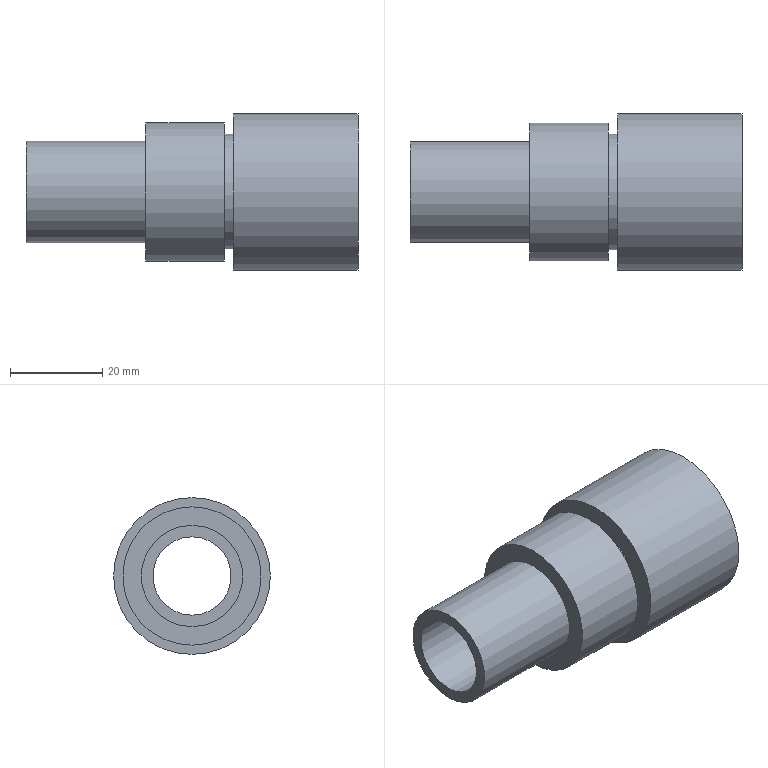Component | NX | SLEEVE | 1 solid | 14 faces | box 72 x 34 x 34 mm | volume 29705 mm3 | cylinder 7 | plane 7 | commonest cylinder face diameters 30 x1 22 x1 34 x1 17 x1 17.5 x1 25 x1 20 x1
STEP:
#1=CARTESIAN_POINT('',(0.,0.,0.));
#2=DIRECTION('',(0.,0.,1.));
#3=DIRECTION('',(1.,0.,0.));
#4=AXIS2_PLACEMENT_3D('',#1,#2,#3);
#5=CARTESIAN_POINT('',(21.,-0.,5.));
#6=VERTEX_POINT('',#5);
#7=CARTESIAN_POINT('',(21.,-0.,20.));
#8=DIRECTION('',(1.,0.,0.));
#9=DIRECTION('',(0.,0.,-1.));
#10=AXIS2_PLACEMENT_3D('',#7,#8,#9);
#11=CIRCLE('',#10,15.);
#12=CARTESIAN_POINT('',(40.,-0.,20.));
#13=DIRECTION('',(-1.,0.,0.));
#14=DIRECTION('',(0.,0.,1.));
#15=AXIS2_PLACEMENT_3D('',#12,#13,#14);
#16=CYLINDRICAL_SURFACE('',#15,15.);
#17=CARTESIAN_POINT('',(9.425,19.));
#18=DIRECTION('',(-1.,0.));
#19=VECTOR('',#18,1.);
#20=LINE('',#17,#19);
#21=(GEOMETRIC_REPRESENTATION_CONTEXT(2)PARAMETRIC_REPRESENTATION_CONTEXT()REPRESENTATION_CONTEXT('',''));
#22=DEFINITIONAL_REPRESENTATION('',(#20),#21);
#23=PCURVE('',#16,#22);
#24=CARTESIAN_POINT('',(21.,-0.,20.));
#25=DIRECTION('',(1.,0.,0.));
#26=DIRECTION('',(0.,0.,-1.));
#27=AXIS2_PLACEMENT_3D('',#24,#25,#26);
#28=PLANE('',#27);
#29=CARTESIAN_POINT('',(0.,0.));
#30=DIRECTION('',(1.,0.));
#31=AXIS2_PLACEMENT_2D('',#29,#30);
#32=CIRCLE('',#31,15.);
#33=(GEOMETRIC_REPRESENTATION_CONTEXT(2)PARAMETRIC_REPRESENTATION_CONTEXT()REPRESENTATION_CONTEXT('',''));
#34=DEFINITIONAL_REPRESENTATION('',(#32),#33);
#35=PCURVE('',#28,#34);
#36=SURFACE_CURVE('',#11,(#23,#35),.PCURVE_S1.);
#37=EDGE_CURVE('',#6,#6,#36,.T.);
#38=ORIENTED_EDGE('',*,*,#37,.T.);
#39=CARTESIAN_POINT('',(38.,-0.,5.));
#40=VERTEX_POINT('',#39);
#41=CARTESIAN_POINT('',(38.,-0.,5.));
#42=CARTESIAN_POINT('',(21.,-0.,5.));
#43=B_SPLINE_CURVE_WITH_KNOTS('',1,(#41,#42),.UNSPECIFIED.,.F.,.F.,(2,2),(2.,19.),.PIECEWISE_BEZIER_KNOTS.);
#44=CARTESIAN_POINT('',(3.142,0.));
#45=DIRECTION('',(0.,1.));
#46=VECTOR('',#45,1.);
#47=LINE('',#44,#46);
#48=(GEOMETRIC_REPRESENTATION_CONTEXT(2)PARAMETRIC_REPRESENTATION_CONTEXT()REPRESENTATION_CONTEXT('',''));
#49=DEFINITIONAL_REPRESENTATION('',(#47),#48);
#50=PCURVE('',#16,#49);
#51=CARTESIAN_POINT('',(9.425,0.));
#52=DIRECTION('',(0.,1.));
#53=VECTOR('',#52,1.);
#54=LINE('',#51,#53);
#55=(GEOMETRIC_REPRESENTATION_CONTEXT(2)PARAMETRIC_REPRESENTATION_CONTEXT()REPRESENTATION_CONTEXT('',''));
#56=DEFINITIONAL_REPRESENTATION('',(#54),#55);
#57=PCURVE('',#16,#56);
#58=SEAM_CURVE('',#43,(#50,#57),.PCURVE_S1.);
#59=EDGE_CURVE('',#40,#6,#58,.T.);
#60=ORIENTED_EDGE('',*,*,#59,.F.);
#61=CARTESIAN_POINT('',(38.,-0.,20.));
#62=DIRECTION('',(1.,0.,0.));
#63=DIRECTION('',(0.,0.,-1.));
#64=AXIS2_PLACEMENT_3D('',#61,#62,#63);
#65=CIRCLE('',#64,15.);
#66=CARTESIAN_POINT('',(9.425,2.));
#67=DIRECTION('',(-1.,0.));
#68=VECTOR('',#67,1.);
#69=LINE('',#66,#68);
#70=(GEOMETRIC_REPRESENTATION_CONTEXT(2)PARAMETRIC_REPRESENTATION_CONTEXT()REPRESENTATION_CONTEXT('',''));
#71=DEFINITIONAL_REPRESENTATION('',(#69),#70);
#72=PCURVE('',#16,#71);
#73=CARTESIAN_POINT('',(38.,-0.,20.));
#74=DIRECTION('',(-1.,0.,0.));
#75=DIRECTION('',(0.,0.,1.));
#76=AXIS2_PLACEMENT_3D('',#73,#74,#75);
#77=PLANE('',#76);
#78=CARTESIAN_POINT('',(-15.,0.));
#79=CARTESIAN_POINT('',(-15.,25.981));
#80=CARTESIAN_POINT('',(7.5,12.99));
#81=CARTESIAN_POINT('',(30.,0.));
#82=CARTESIAN_POINT('',(7.5,-12.99));
#83=CARTESIAN_POINT('',(-15.,-25.981));
#84=CARTESIAN_POINT('',(-15.,0.));
#85=(BOUNDED_CURVE()B_SPLINE_CURVE(2,(#78,#79,#80,#81,#82,#83,#84),.UNSPECIFIED.,.T.,.F.)B_SPLINE_CURVE_WITH_KNOTS((1,2,2,2,2,1),(-2.094,0.,2.094,4.189,6.283,8.378),.UNSPECIFIED.)CURVE()GEOMETRIC_REPRESENTATION_ITEM()RATIONAL_B_SPLINE_CURVE((1.,0.5,1.,0.5,1.,0.5,1.))REPRESENTATION_ITEM(''));
#86=(GEOMETRIC_REPRESENTATION_CONTEXT(2)PARAMETRIC_REPRESENTATION_CONTEXT()REPRESENTATION_CONTEXT('',''));
#87=DEFINITIONAL_REPRESENTATION('',(#85),#86);
#88=PCURVE('',#77,#87);
#89=SURFACE_CURVE('',#65,(#72,#88),.PCURVE_S1.);
#90=EDGE_CURVE('',#40,#40,#89,.T.);
#91=ORIENTED_EDGE('',*,*,#90,.F.);
#92=ORIENTED_EDGE('',*,*,#59,.T.);
#93=EDGE_LOOP('',(#38,#60,#91,#92));
#94=FACE_BOUND('',#93,.T.);
#95=ADVANCED_FACE('',(#94),#16,.T.);
#96=CARTESIAN_POINT('',(21.,-0.,9.));
#97=VERTEX_POINT('',#96);
#98=CARTESIAN_POINT('',(21.,-0.,20.));
#99=DIRECTION('',(1.,0.,0.));
#100=DIRECTION('',(0.,0.,-1.));
#101=AXIS2_PLACEMENT_3D('',#98,#99,#100);
#102=CIRCLE('',#101,11.);
#103=CARTESIAN_POINT('',(21.,-0.,20.));
#104=DIRECTION('',(-1.,0.,0.));
#105=DIRECTION('',(0.,0.,1.));
#106=AXIS2_PLACEMENT_3D('',#103,#104,#105);
#107=CYLINDRICAL_SURFACE('',#106,11.);
#108=CARTESIAN_POINT('',(9.425,0.));
#109=DIRECTION('',(-1.,0.));
#110=VECTOR('',#109,1.);
#111=LINE('',#108,#110);
#112=(GEOMETRIC_REPRESENTATION_CONTEXT(2)PARAMETRIC_REPRESENTATION_CONTEXT()REPRESENTATION_CONTEXT('',''));
#113=DEFINITIONAL_REPRESENTATION('',(#111),#112);
#114=PCURVE('',#107,#113);
#115=CARTESIAN_POINT('',(0.,0.));
#116=DIRECTION('',(1.,0.));
#117=AXIS2_PLACEMENT_2D('',#115,#116);
#118=CIRCLE('',#117,11.);
#119=(GEOMETRIC_REPRESENTATION_CONTEXT(2)PARAMETRIC_REPRESENTATION_CONTEXT()REPRESENTATION_CONTEXT('',''));
#120=DEFINITIONAL_REPRESENTATION('',(#118),#119);
#121=PCURVE('',#28,#120);
#122=SURFACE_CURVE('',#102,(#114,#121),.PCURVE_S1.);
#123=EDGE_CURVE('',#97,#97,#122,.T.);
#124=ORIENTED_EDGE('',*,*,#123,.F.);
#125=CARTESIAN_POINT('',(-5.,-0.,9.));
#126=VERTEX_POINT('',#125);
#127=CARTESIAN_POINT('',(21.,-0.,9.));
#128=CARTESIAN_POINT('',(-5.,-0.,9.));
#129=B_SPLINE_CURVE_WITH_KNOTS('',1,(#127,#128),.UNSPECIFIED.,.F.,.F.,(2,2),(0.,26.),.PIECEWISE_BEZIER_KNOTS.);
#130=CARTESIAN_POINT('',(9.425,0.));
#131=DIRECTION('',(0.,1.));
#132=VECTOR('',#131,1.);
#133=LINE('',#130,#132);
#134=(GEOMETRIC_REPRESENTATION_CONTEXT(2)PARAMETRIC_REPRESENTATION_CONTEXT()REPRESENTATION_CONTEXT('',''));
#135=DEFINITIONAL_REPRESENTATION('',(#133),#134);
#136=PCURVE('',#107,#135);
#137=CARTESIAN_POINT('',(3.142,0.));
#138=DIRECTION('',(0.,1.));
#139=VECTOR('',#138,1.);
#140=LINE('',#137,#139);
#141=(GEOMETRIC_REPRESENTATION_CONTEXT(2)PARAMETRIC_REPRESENTATION_CONTEXT()REPRESENTATION_CONTEXT('',''));
#142=DEFINITIONAL_REPRESENTATION('',(#140),#141);
#143=PCURVE('',#107,#142);
#144=SEAM_CURVE('',#129,(#136,#143),.PCURVE_S1.);
#145=EDGE_CURVE('',#97,#126,#144,.T.);
#146=ORIENTED_EDGE('',*,*,#145,.T.);
#147=CARTESIAN_POINT('',(-5.,-0.,20.));
#148=DIRECTION('',(1.,0.,0.));
#149=DIRECTION('',(0.,0.,-1.));
#150=AXIS2_PLACEMENT_3D('',#147,#148,#149);
#151=CIRCLE('',#150,11.);
#152=CARTESIAN_POINT('',(9.425,26.));
#153=DIRECTION('',(-1.,0.));
#154=VECTOR('',#153,1.);
#155=LINE('',#152,#154);
#156=(GEOMETRIC_REPRESENTATION_CONTEXT(2)PARAMETRIC_REPRESENTATION_CONTEXT()REPRESENTATION_CONTEXT('',''));
#157=DEFINITIONAL_REPRESENTATION('',(#155),#156);
#158=PCURVE('',#107,#157);
#159=CARTESIAN_POINT('',(-5.,-0.,20.));
#160=DIRECTION('',(1.,0.,0.));
#161=DIRECTION('',(0.,0.,-1.));
#162=AXIS2_PLACEMENT_3D('',#159,#160,#161);
#163=PLANE('',#162);
#164=CARTESIAN_POINT('',(0.,0.));
#165=DIRECTION('',(1.,0.));
#166=AXIS2_PLACEMENT_2D('',#164,#165);
#167=CIRCLE('',#166,11.);
#168=(GEOMETRIC_REPRESENTATION_CONTEXT(2)PARAMETRIC_REPRESENTATION_CONTEXT()REPRESENTATION_CONTEXT('',''));
#169=DEFINITIONAL_REPRESENTATION('',(#167),#168);
#170=PCURVE('',#163,#169);
#171=SURFACE_CURVE('',#151,(#158,#170),.PCURVE_S1.);
#172=EDGE_CURVE('',#126,#126,#171,.T.);
#173=ORIENTED_EDGE('',*,*,#172,.T.);
#174=ORIENTED_EDGE('',*,*,#145,.F.);
#175=EDGE_LOOP('',(#124,#146,#173,#174));
#176=FACE_BOUND('',#175,.T.);
#177=ADVANCED_FACE('',(#176),#107,.T.);
#178=CARTESIAN_POINT('',(-5.,-0.,11.5));
#179=VERTEX_POINT('',#178);
#180=CARTESIAN_POINT('',(-5.,-0.,20.));
#181=DIRECTION('',(1.,0.,0.));
#182=DIRECTION('',(0.,0.,-1.));
#183=AXIS2_PLACEMENT_3D('',#180,#181,#182);
#184=CIRCLE('',#183,8.5);
#185=CARTESIAN_POINT('',(0.,0.));
#186=DIRECTION('',(1.,0.));
#187=AXIS2_PLACEMENT_2D('',#185,#186);
#188=CIRCLE('',#187,8.5);
#189=(GEOMETRIC_REPRESENTATION_CONTEXT(2)PARAMETRIC_REPRESENTATION_CONTEXT()REPRESENTATION_CONTEXT('',''));
#190=DEFINITIONAL_REPRESENTATION('',(#188),#189);
#191=PCURVE('',#163,#190);
#192=CARTESIAN_POINT('',(-5.,-0.,20.));
#193=DIRECTION('',(1.,0.,0.));
#194=DIRECTION('',(0.,0.,-1.));
#195=AXIS2_PLACEMENT_3D('',#192,#193,#194);
#196=CYLINDRICAL_SURFACE('',#195,8.5);
#197=CARTESIAN_POINT('',(0.,0.));
#198=DIRECTION('',(1.,0.));
#199=VECTOR('',#198,1.);
#200=LINE('',#197,#199);
#201=(GEOMETRIC_REPRESENTATION_CONTEXT(2)PARAMETRIC_REPRESENTATION_CONTEXT()REPRESENTATION_CONTEXT('',''));
#202=DEFINITIONAL_REPRESENTATION('',(#200),#201);
#203=PCURVE('',#196,#202);
#204=SURFACE_CURVE('',#184,(#191,#203),.PCURVE_S1.);
#205=EDGE_CURVE('',#179,#179,#204,.T.);
#206=ORIENTED_EDGE('',*,*,#205,.T.);
#207=EDGE_LOOP('',(#206));
#208=FACE_BOUND('',#207,.T.);
#209=ORIENTED_EDGE('',*,*,#172,.F.);
#210=EDGE_LOOP('',(#209));
#211=FACE_BOUND('',#210,.T.);
#212=ADVANCED_FACE('',(#208,#211),#163,.F.);
#213=ORIENTED_EDGE('',*,*,#123,.T.);
#214=EDGE_LOOP('',(#213));
#215=FACE_BOUND('',#214,.T.);
#216=ORIENTED_EDGE('',*,*,#37,.F.);
#217=EDGE_LOOP('',(#216));
#218=FACE_BOUND('',#217,.T.);
#219=ADVANCED_FACE('',(#215,#218),#28,.F.);
#220=CARTESIAN_POINT('',(67.,-0.,3.));
#221=VERTEX_POINT('',#220);
#222=CARTESIAN_POINT('',(67.,-0.,20.));
#223=DIRECTION('',(1.,0.,0.));
#224=DIRECTION('',(0.,0.,-1.));
#225=AXIS2_PLACEMENT_3D('',#222,#223,#224);
#226=CIRCLE('',#225,17.);
#227=CARTESIAN_POINT('',(67.,-0.,20.));
#228=DIRECTION('',(-1.,0.,0.));
#229=DIRECTION('',(0.,0.,1.));
#230=AXIS2_PLACEMENT_3D('',#227,#228,#229);
#231=CYLINDRICAL_SURFACE('',#230,17.);
#232=CARTESIAN_POINT('',(9.425,0.));
#233=DIRECTION('',(-1.,0.));
#234=VECTOR('',#233,1.);
#235=LINE('',#232,#234);
#236=(GEOMETRIC_REPRESENTATION_CONTEXT(2)PARAMETRIC_REPRESENTATION_CONTEXT()REPRESENTATION_CONTEXT('',''));
#237=DEFINITIONAL_REPRESENTATION('',(#235),#236);
#238=PCURVE('',#231,#237);
#239=CARTESIAN_POINT('',(67.,-0.,20.));
#240=DIRECTION('',(1.,0.,0.));
#241=DIRECTION('',(0.,0.,-1.));
#242=AXIS2_PLACEMENT_3D('',#239,#240,#241);
#243=PLANE('',#242);
#244=CARTESIAN_POINT('',(0.,0.));
#245=DIRECTION('',(1.,0.));
#246=AXIS2_PLACEMENT_2D('',#244,#245);
#247=CIRCLE('',#246,17.);
#248=(GEOMETRIC_REPRESENTATION_CONTEXT(2)PARAMETRIC_REPRESENTATION_CONTEXT()REPRESENTATION_CONTEXT('',''));
#249=DEFINITIONAL_REPRESENTATION('',(#247),#248);
#250=PCURVE('',#243,#249);
#251=SURFACE_CURVE('',#226,(#238,#250),.PCURVE_S1.);
#252=EDGE_CURVE('',#221,#221,#251,.T.);
#253=ORIENTED_EDGE('',*,*,#252,.F.);
#254=CARTESIAN_POINT('',(40.,-0.,3.));
#255=VERTEX_POINT('',#254);
#256=CARTESIAN_POINT('',(67.,-0.,3.));
#257=CARTESIAN_POINT('',(40.,-0.,3.));
#258=B_SPLINE_CURVE_WITH_KNOTS('',1,(#256,#257),.UNSPECIFIED.,.F.,.F.,(2,2),(0.,27.),.PIECEWISE_BEZIER_KNOTS.);
#259=CARTESIAN_POINT('',(9.425,0.));
#260=DIRECTION('',(0.,1.));
#261=VECTOR('',#260,1.);
#262=LINE('',#259,#261);
#263=(GEOMETRIC_REPRESENTATION_CONTEXT(2)PARAMETRIC_REPRESENTATION_CONTEXT()REPRESENTATION_CONTEXT('',''));
#264=DEFINITIONAL_REPRESENTATION('',(#262),#263);
#265=PCURVE('',#231,#264);
#266=CARTESIAN_POINT('',(3.142,0.));
#267=DIRECTION('',(0.,1.));
#268=VECTOR('',#267,1.);
#269=LINE('',#266,#268);
#270=(GEOMETRIC_REPRESENTATION_CONTEXT(2)PARAMETRIC_REPRESENTATION_CONTEXT()REPRESENTATION_CONTEXT('',''));
#271=DEFINITIONAL_REPRESENTATION('',(#269),#270);
#272=PCURVE('',#231,#271);
#273=SEAM_CURVE('',#258,(#265,#272),.PCURVE_S1.);
#274=EDGE_CURVE('',#221,#255,#273,.T.);
#275=ORIENTED_EDGE('',*,*,#274,.T.);
#276=CARTESIAN_POINT('',(40.,-0.,20.));
#277=DIRECTION('',(1.,0.,0.));
#278=DIRECTION('',(0.,0.,-1.));
#279=AXIS2_PLACEMENT_3D('',#276,#277,#278);
#280=CIRCLE('',#279,17.);
#281=CARTESIAN_POINT('',(9.425,27.));
#282=DIRECTION('',(-1.,0.));
#283=VECTOR('',#282,1.);
#284=LINE('',#281,#283);
#285=(GEOMETRIC_REPRESENTATION_CONTEXT(2)PARAMETRIC_REPRESENTATION_CONTEXT()REPRESENTATION_CONTEXT('',''));
#286=DEFINITIONAL_REPRESENTATION('',(#284),#285);
#287=PCURVE('',#231,#286);
#288=CARTESIAN_POINT('',(40.,-0.,20.));
#289=DIRECTION('',(1.,0.,0.));
#290=DIRECTION('',(0.,0.,-1.));
#291=AXIS2_PLACEMENT_3D('',#288,#289,#290);
#292=PLANE('',#291);
#293=CARTESIAN_POINT('',(0.,0.));
#294=DIRECTION('',(1.,0.));
#295=AXIS2_PLACEMENT_2D('',#293,#294);
#296=CIRCLE('',#295,17.);
#297=(GEOMETRIC_REPRESENTATION_CONTEXT(2)PARAMETRIC_REPRESENTATION_CONTEXT()REPRESENTATION_CONTEXT('',''));
#298=DEFINITIONAL_REPRESENTATION('',(#296),#297);
#299=PCURVE('',#292,#298);
#300=SURFACE_CURVE('',#280,(#287,#299),.PCURVE_S1.);
#301=EDGE_CURVE('',#255,#255,#300,.T.);
#302=ORIENTED_EDGE('',*,*,#301,.T.);
#303=ORIENTED_EDGE('',*,*,#274,.F.);
#304=EDGE_LOOP('',(#253,#275,#302,#303));
#305=FACE_BOUND('',#304,.T.);
#306=ADVANCED_FACE('',(#305),#231,.T.);
#307=CARTESIAN_POINT('',(67.,-0.,10.));
#308=VERTEX_POINT('',#307);
#309=CARTESIAN_POINT('',(67.,-0.,20.));
#310=DIRECTION('',(1.,0.,0.));
#311=DIRECTION('',(0.,0.,-1.));
#312=AXIS2_PLACEMENT_3D('',#309,#310,#311);
#313=CIRCLE('',#312,10.);
#314=CARTESIAN_POINT('',(0.,0.));
#315=DIRECTION('',(1.,0.));
#316=AXIS2_PLACEMENT_2D('',#314,#315);
#317=CIRCLE('',#316,10.);
#318=(GEOMETRIC_REPRESENTATION_CONTEXT(2)PARAMETRIC_REPRESENTATION_CONTEXT()REPRESENTATION_CONTEXT('',''));
#319=DEFINITIONAL_REPRESENTATION('',(#317),#318);
#320=PCURVE('',#243,#319);
#321=CARTESIAN_POINT('',(52.,-0.,20.));
#322=DIRECTION('',(1.,0.,0.));
#323=DIRECTION('',(0.,0.,-1.));
#324=AXIS2_PLACEMENT_3D('',#321,#322,#323);
#325=CYLINDRICAL_SURFACE('',#324,10.);
#326=CARTESIAN_POINT('',(0.,15.));
#327=DIRECTION('',(1.,0.));
#328=VECTOR('',#327,1.);
#329=LINE('',#326,#328);
#330=(GEOMETRIC_REPRESENTATION_CONTEXT(2)PARAMETRIC_REPRESENTATION_CONTEXT()REPRESENTATION_CONTEXT('',''));
#331=DEFINITIONAL_REPRESENTATION('',(#329),#330);
#332=PCURVE('',#325,#331);
#333=SURFACE_CURVE('',#313,(#320,#332),.PCURVE_S1.);
#334=EDGE_CURVE('',#308,#308,#333,.T.);
#335=ORIENTED_EDGE('',*,*,#334,.F.);
#336=EDGE_LOOP('',(#335));
#337=FACE_BOUND('',#336,.T.);
#338=ORIENTED_EDGE('',*,*,#252,.T.);
#339=EDGE_LOOP('',(#338));
#340=FACE_BOUND('',#339,.T.);
#341=ADVANCED_FACE('',(#337,#340),#243,.T.);
#342=ORIENTED_EDGE('',*,*,#301,.F.);
#343=EDGE_LOOP('',(#342));
#344=FACE_BOUND('',#343,.T.);
#345=CARTESIAN_POINT('',(40.,-0.,32.5));
#346=VERTEX_POINT('',#345);
#347=CARTESIAN_POINT('',(40.,-0.,20.));
#348=DIRECTION('',(1.,0.,0.));
#349=DIRECTION('',(0.,0.,1.));
#350=AXIS2_PLACEMENT_3D('',#347,#348,#349);
#351=CIRCLE('',#350,12.5);
#352=CARTESIAN_POINT('',(0.,0.));
#353=DIRECTION('',(-1.,0.));
#354=AXIS2_PLACEMENT_2D('',#352,#353);
#355=CIRCLE('',#354,12.5);
#356=(GEOMETRIC_REPRESENTATION_CONTEXT(2)PARAMETRIC_REPRESENTATION_CONTEXT()REPRESENTATION_CONTEXT('',''));
#357=DEFINITIONAL_REPRESENTATION('',(#355),#356);
#358=PCURVE('',#292,#357);
#359=CARTESIAN_POINT('',(40.,-0.,20.));
#360=DIRECTION('',(-1.,0.,0.));
#361=DIRECTION('',(0.,0.,1.));
#362=AXIS2_PLACEMENT_3D('',#359,#360,#361);
#363=CYLINDRICAL_SURFACE('',#362,12.5);
#364=CARTESIAN_POINT('',(6.283,0.));
#365=DIRECTION('',(-1.,0.));
#366=VECTOR('',#365,1.);
#367=LINE('',#364,#366);
#368=(GEOMETRIC_REPRESENTATION_CONTEXT(2)PARAMETRIC_REPRESENTATION_CONTEXT()REPRESENTATION_CONTEXT('',''));
#369=DEFINITIONAL_REPRESENTATION('',(#367),#368);
#370=PCURVE('',#363,#369);
#371=SURFACE_CURVE('',#351,(#358,#370),.PCURVE_S1.);
#372=EDGE_CURVE('',#346,#346,#371,.T.);
#373=ORIENTED_EDGE('',*,*,#372,.T.);
#374=EDGE_LOOP('',(#373));
#375=FACE_BOUND('',#374,.T.);
#376=ADVANCED_FACE('',(#344,#375),#292,.F.);
#377=CARTESIAN_POINT('',(49.,-0.,11.5));
#378=VERTEX_POINT('',#377);
#379=CARTESIAN_POINT('',(49.,-0.,28.5));
#380=VERTEX_POINT('',#379);
#381=CARTESIAN_POINT('',(49.,-0.,20.));
#382=DIRECTION('',(1.,0.,0.));
#383=DIRECTION('',(0.,0.,1.));
#384=AXIS2_PLACEMENT_3D('',#381,#382,#383);
#385=CIRCLE('',#384,8.5);
#386=CARTESIAN_POINT('',(-3.142,54.));
#387=DIRECTION('',(1.,0.));
#388=VECTOR('',#387,1.);
#389=LINE('',#386,#388);
#390=(GEOMETRIC_REPRESENTATION_CONTEXT(2)PARAMETRIC_REPRESENTATION_CONTEXT()REPRESENTATION_CONTEXT('',''));
#391=DEFINITIONAL_REPRESENTATION('',(#389),#390);
#392=PCURVE('',#196,#391);
#393=CARTESIAN_POINT('',(49.,-0.,20.));
#394=DIRECTION('',(-1.,0.,0.));
#395=DIRECTION('',(0.,0.,1.));
#396=AXIS2_PLACEMENT_3D('',#393,#394,#395);
#397=PLANE('',#396);
#398=CARTESIAN_POINT('',(8.5,0.));
#399=CARTESIAN_POINT('',(8.5,-14.722));
#400=CARTESIAN_POINT('',(-4.25,-7.361));
#401=CARTESIAN_POINT('',(-17.,-0.));
#402=CARTESIAN_POINT('',(-4.25,7.361));
#403=CARTESIAN_POINT('',(8.5,14.722));
#404=CARTESIAN_POINT('',(8.5,0.));
#405=(BOUNDED_CURVE()B_SPLINE_CURVE(2,(#398,#399,#400,#401,#402,#403,#404),.UNSPECIFIED.,.T.,.F.)B_SPLINE_CURVE_WITH_KNOTS((1,2,2,2,2,1),(-2.094,0.,2.094,4.189,6.283,8.378),.UNSPECIFIED.)CURVE()GEOMETRIC_REPRESENTATION_ITEM()RATIONAL_B_SPLINE_CURVE((1.,0.5,1.,0.5,1.,0.5,1.))REPRESENTATION_ITEM(''));
#406=(GEOMETRIC_REPRESENTATION_CONTEXT(2)PARAMETRIC_REPRESENTATION_CONTEXT()REPRESENTATION_CONTEXT('',''));
#407=DEFINITIONAL_REPRESENTATION('',(#405),#406);
#408=PCURVE('',#397,#407);
#409=SURFACE_CURVE('',#385,(#392,#408),.PCURVE_S1.);
#410=EDGE_CURVE('',#378,#380,#409,.T.);
#411=ORIENTED_EDGE('',*,*,#410,.F.);
#412=CARTESIAN_POINT('',(-5.,-0.,11.5));
#413=CARTESIAN_POINT('',(49.,-0.,11.5));
#414=B_SPLINE_CURVE_WITH_KNOTS('',1,(#412,#413),.UNSPECIFIED.,.F.,.F.,(2,2),(0.,54.),.PIECEWISE_BEZIER_KNOTS.);
#415=CARTESIAN_POINT('',(0.,0.));
#416=DIRECTION('',(0.,1.));
#417=VECTOR('',#416,1.);
#418=LINE('',#415,#417);
#419=(GEOMETRIC_REPRESENTATION_CONTEXT(2)PARAMETRIC_REPRESENTATION_CONTEXT()REPRESENTATION_CONTEXT('',''));
#420=DEFINITIONAL_REPRESENTATION('',(#418),#419);
#421=PCURVE('',#196,#420);
#422=CARTESIAN_POINT('',(6.283,0.));
#423=DIRECTION('',(0.,1.));
#424=VECTOR('',#423,1.);
#425=LINE('',#422,#424);
#426=(GEOMETRIC_REPRESENTATION_CONTEXT(2)PARAMETRIC_REPRESENTATION_CONTEXT()REPRESENTATION_CONTEXT('',''));
#427=DEFINITIONAL_REPRESENTATION('',(#425),#426);
#428=PCURVE('',#196,#427);
#429=SEAM_CURVE('',#414,(#421,#428),.PCURVE_S1.);
#430=EDGE_CURVE('',#179,#378,#429,.T.);
#431=ORIENTED_EDGE('',*,*,#430,.F.);
#432=ORIENTED_EDGE('',*,*,#205,.T.);
#433=ORIENTED_EDGE('',*,*,#430,.T.);
#434=CARTESIAN_POINT('',(49.,-0.,20.));
#435=DIRECTION('',(1.,0.,0.));
#436=DIRECTION('',(0.,0.,1.));
#437=AXIS2_PLACEMENT_3D('',#434,#435,#436);
#438=CIRCLE('',#437,8.5);
#439=CARTESIAN_POINT('',(3.142,54.));
#440=DIRECTION('',(1.,0.));
#441=VECTOR('',#440,1.);
#442=LINE('',#439,#441);
#443=(GEOMETRIC_REPRESENTATION_CONTEXT(2)PARAMETRIC_REPRESENTATION_CONTEXT()REPRESENTATION_CONTEXT('',''));
#444=DEFINITIONAL_REPRESENTATION('',(#442),#443);
#445=PCURVE('',#196,#444);
#446=CARTESIAN_POINT('',(8.5,0.));
#447=CARTESIAN_POINT('',(8.5,-14.722));
#448=CARTESIAN_POINT('',(-4.25,-7.361));
#449=CARTESIAN_POINT('',(-17.,-0.));
#450=CARTESIAN_POINT('',(-4.25,7.361));
#451=CARTESIAN_POINT('',(8.5,14.722));
#452=CARTESIAN_POINT('',(8.5,0.));
#453=(BOUNDED_CURVE()B_SPLINE_CURVE(2,(#446,#447,#448,#449,#450,#451,#452),.UNSPECIFIED.,.T.,.F.)B_SPLINE_CURVE_WITH_KNOTS((1,2,2,2,2,1),(-2.094,0.,2.094,4.189,6.283,8.378),.UNSPECIFIED.)CURVE()GEOMETRIC_REPRESENTATION_ITEM()RATIONAL_B_SPLINE_CURVE((1.,0.5,1.,0.5,1.,0.5,1.))REPRESENTATION_ITEM(''));
#454=(GEOMETRIC_REPRESENTATION_CONTEXT(2)PARAMETRIC_REPRESENTATION_CONTEXT()REPRESENTATION_CONTEXT('',''));
#455=DEFINITIONAL_REPRESENTATION('',(#453),#454);
#456=PCURVE('',#397,#455);
#457=SURFACE_CURVE('',#438,(#445,#456),.PCURVE_S1.);
#458=EDGE_CURVE('',#380,#378,#457,.T.);
#459=ORIENTED_EDGE('',*,*,#458,.F.);
#460=EDGE_LOOP('',(#411,#431,#432,#433,#459));
#461=FACE_BOUND('',#460,.F.);
#462=ADVANCED_FACE('',(#461),#196,.F.);
#463=CARTESIAN_POINT('',(49.,-0.,28.75));
#464=VERTEX_POINT('',#463);
#465=CARTESIAN_POINT('',(49.,-0.,20.));
#466=DIRECTION('',(1.,0.,0.));
#467=DIRECTION('',(0.,0.,1.));
#468=AXIS2_PLACEMENT_3D('',#465,#466,#467);
#469=CIRCLE('',#468,8.75);
#470=CARTESIAN_POINT('',(8.75,0.));
#471=CARTESIAN_POINT('',(8.75,-15.155));
#472=CARTESIAN_POINT('',(-4.375,-7.578));
#473=CARTESIAN_POINT('',(-17.5,-0.));
#474=CARTESIAN_POINT('',(-4.375,7.578));
#475=CARTESIAN_POINT('',(8.75,15.155));
#476=CARTESIAN_POINT('',(8.75,0.));
#477=(BOUNDED_CURVE()B_SPLINE_CURVE(2,(#470,#471,#472,#473,#474,#475,#476),.UNSPECIFIED.,.T.,.F.)B_SPLINE_CURVE_WITH_KNOTS((1,2,2,2,2,1),(-2.094,0.,2.094,4.189,6.283,8.378),.UNSPECIFIED.)CURVE()GEOMETRIC_REPRESENTATION_ITEM()RATIONAL_B_SPLINE_CURVE((1.,0.5,1.,0.5,1.,0.5,1.))REPRESENTATION_ITEM(''));
#478=(GEOMETRIC_REPRESENTATION_CONTEXT(2)PARAMETRIC_REPRESENTATION_CONTEXT()REPRESENTATION_CONTEXT('',''));
#479=DEFINITIONAL_REPRESENTATION('',(#477),#478);
#480=PCURVE('',#397,#479);
#481=CARTESIAN_POINT('',(67.,-0.,20.));
#482=DIRECTION('',(-1.,0.,0.));
#483=DIRECTION('',(0.,0.,1.));
#484=AXIS2_PLACEMENT_3D('',#481,#482,#483);
#485=CYLINDRICAL_SURFACE('',#484,8.75);
#486=CARTESIAN_POINT('',(6.283,18.));
#487=DIRECTION('',(-1.,0.));
#488=VECTOR('',#487,1.);
#489=LINE('',#486,#488);
#490=(GEOMETRIC_REPRESENTATION_CONTEXT(2)PARAMETRIC_REPRESENTATION_CONTEXT()REPRESENTATION_CONTEXT('',''));
#491=DEFINITIONAL_REPRESENTATION('',(#489),#490);
#492=PCURVE('',#485,#491);
#493=SURFACE_CURVE('',#469,(#480,#492),.PCURVE_S1.);
#494=EDGE_CURVE('',#464,#464,#493,.T.);
#495=ORIENTED_EDGE('',*,*,#494,.T.);
#496=EDGE_LOOP('',(#495));
#497=FACE_BOUND('',#496,.T.);
#498=ORIENTED_EDGE('',*,*,#458,.F.);
#499=ORIENTED_EDGE('',*,*,#410,.F.);
#500=EDGE_LOOP('',(#498,#499));
#501=FACE_BOUND('',#500,.T.);
#502=ADVANCED_FACE('',(#497,#501),#397,.F.);
#503=CARTESIAN_POINT('',(52.,-0.,28.75));
#504=VERTEX_POINT('',#503);
#505=CARTESIAN_POINT('',(52.,-0.,20.));
#506=DIRECTION('',(1.,0.,0.));
#507=DIRECTION('',(0.,0.,1.));
#508=AXIS2_PLACEMENT_3D('',#505,#506,#507);
#509=CIRCLE('',#508,8.75);
#510=CARTESIAN_POINT('',(6.283,15.));
#511=DIRECTION('',(-1.,0.));
#512=VECTOR('',#511,1.);
#513=LINE('',#510,#512);
#514=(GEOMETRIC_REPRESENTATION_CONTEXT(2)PARAMETRIC_REPRESENTATION_CONTEXT()REPRESENTATION_CONTEXT('',''));
#515=DEFINITIONAL_REPRESENTATION('',(#513),#514);
#516=PCURVE('',#485,#515);
#517=CARTESIAN_POINT('',(52.,-0.,20.));
#518=DIRECTION('',(-1.,0.,0.));
#519=DIRECTION('',(0.,0.,1.));
#520=AXIS2_PLACEMENT_3D('',#517,#518,#519);
#521=PLANE('',#520);
#522=CARTESIAN_POINT('',(8.75,0.));
#523=CARTESIAN_POINT('',(8.75,-15.155));
#524=CARTESIAN_POINT('',(-4.375,-7.578));
#525=CARTESIAN_POINT('',(-17.5,-0.));
#526=CARTESIAN_POINT('',(-4.375,7.578));
#527=CARTESIAN_POINT('',(8.75,15.155));
#528=CARTESIAN_POINT('',(8.75,0.));
#529=(BOUNDED_CURVE()B_SPLINE_CURVE(2,(#522,#523,#524,#525,#526,#527,#528),.UNSPECIFIED.,.T.,.F.)B_SPLINE_CURVE_WITH_KNOTS((1,2,2,2,2,1),(-2.094,0.,2.094,4.189,6.283,8.378),.UNSPECIFIED.)CURVE()GEOMETRIC_REPRESENTATION_ITEM()RATIONAL_B_SPLINE_CURVE((1.,0.5,1.,0.5,1.,0.5,1.))REPRESENTATION_ITEM(''));
#530=(GEOMETRIC_REPRESENTATION_CONTEXT(2)PARAMETRIC_REPRESENTATION_CONTEXT()REPRESENTATION_CONTEXT('',''));
#531=DEFINITIONAL_REPRESENTATION('',(#529),#530);
#532=PCURVE('',#521,#531);
#533=SURFACE_CURVE('',#509,(#516,#532),.PCURVE_S1.);
#534=EDGE_CURVE('',#504,#504,#533,.T.);
#535=ORIENTED_EDGE('',*,*,#534,.F.);
#536=CARTESIAN_POINT('',(52.,-0.,28.75));
#537=CARTESIAN_POINT('',(49.,-0.,28.75));
#538=B_SPLINE_CURVE_WITH_KNOTS('',1,(#536,#537),.UNSPECIFIED.,.F.,.F.,(2,2),(15.,18.),.PIECEWISE_BEZIER_KNOTS.);
#539=CARTESIAN_POINT('',(6.283,0.));
#540=DIRECTION('',(0.,1.));
#541=VECTOR('',#540,1.);
#542=LINE('',#539,#541);
#543=(GEOMETRIC_REPRESENTATION_CONTEXT(2)PARAMETRIC_REPRESENTATION_CONTEXT()REPRESENTATION_CONTEXT('',''));
#544=DEFINITIONAL_REPRESENTATION('',(#542),#543);
#545=PCURVE('',#485,#544);
#546=CARTESIAN_POINT('',(0.,0.));
#547=DIRECTION('',(0.,1.));
#548=VECTOR('',#547,1.);
#549=LINE('',#546,#548);
#550=(GEOMETRIC_REPRESENTATION_CONTEXT(2)PARAMETRIC_REPRESENTATION_CONTEXT()REPRESENTATION_CONTEXT('',''));
#551=DEFINITIONAL_REPRESENTATION('',(#549),#550);
#552=PCURVE('',#485,#551);
#553=SEAM_CURVE('',#538,(#545,#552),.PCURVE_S1.);
#554=EDGE_CURVE('',#504,#464,#553,.T.);
#555=ORIENTED_EDGE('',*,*,#554,.T.);
#556=ORIENTED_EDGE('',*,*,#494,.T.);
#557=ORIENTED_EDGE('',*,*,#554,.F.);
#558=EDGE_LOOP('',(#535,#555,#556,#557));
#559=FACE_BOUND('',#558,.F.);
#560=ADVANCED_FACE('',(#559),#485,.F.);
#561=CARTESIAN_POINT('',(38.,-0.,32.5));
#562=VERTEX_POINT('',#561);
#563=CARTESIAN_POINT('',(38.,-0.,20.));
#564=DIRECTION('',(-1.,0.,0.));
#565=DIRECTION('',(0.,0.,1.));
#566=AXIS2_PLACEMENT_3D('',#563,#564,#565);
#567=CIRCLE('',#566,12.5);
#568=CARTESIAN_POINT('',(0.,0.));
#569=DIRECTION('',(1.,0.));
#570=AXIS2_PLACEMENT_2D('',#568,#569);
#571=CIRCLE('',#570,12.5);
#572=(GEOMETRIC_REPRESENTATION_CONTEXT(2)PARAMETRIC_REPRESENTATION_CONTEXT()REPRESENTATION_CONTEXT('',''));
#573=DEFINITIONAL_REPRESENTATION('',(#571),#572);
#574=PCURVE('',#77,#573);
#575=CARTESIAN_POINT('',(0.,2.));
#576=DIRECTION('',(1.,0.));
#577=VECTOR('',#576,1.);
#578=LINE('',#575,#577);
#579=(GEOMETRIC_REPRESENTATION_CONTEXT(2)PARAMETRIC_REPRESENTATION_CONTEXT()REPRESENTATION_CONTEXT('',''));
#580=DEFINITIONAL_REPRESENTATION('',(#578),#579);
#581=PCURVE('',#363,#580);
#582=SURFACE_CURVE('',#567,(#574,#581),.PCURVE_S1.);
#583=EDGE_CURVE('',#562,#562,#582,.T.);
#584=ORIENTED_EDGE('',*,*,#583,.T.);
#585=EDGE_LOOP('',(#584));
#586=FACE_BOUND('',#585,.T.);
#587=ORIENTED_EDGE('',*,*,#90,.T.);
#588=EDGE_LOOP('',(#587));
#589=FACE_BOUND('',#588,.T.);
#590=ADVANCED_FACE('',(#586,#589),#77,.F.);
#591=ORIENTED_EDGE('',*,*,#372,.F.);
#592=CARTESIAN_POINT('',(40.,-0.,32.5));
#593=CARTESIAN_POINT('',(38.,-0.,32.5));
#594=B_SPLINE_CURVE_WITH_KNOTS('',1,(#592,#593),.UNSPECIFIED.,.F.,.F.,(2,2),(0.,2.),.PIECEWISE_BEZIER_KNOTS.);
#595=CARTESIAN_POINT('',(6.283,0.));
#596=DIRECTION('',(0.,1.));
#597=VECTOR('',#596,1.);
#598=LINE('',#595,#597);
#599=(GEOMETRIC_REPRESENTATION_CONTEXT(2)PARAMETRIC_REPRESENTATION_CONTEXT()REPRESENTATION_CONTEXT('',''));
#600=DEFINITIONAL_REPRESENTATION('',(#598),#599);
#601=PCURVE('',#363,#600);
#602=CARTESIAN_POINT('',(0.,0.));
#603=DIRECTION('',(0.,1.));
#604=VECTOR('',#603,1.);
#605=LINE('',#602,#604);
#606=(GEOMETRIC_REPRESENTATION_CONTEXT(2)PARAMETRIC_REPRESENTATION_CONTEXT()REPRESENTATION_CONTEXT('',''));
#607=DEFINITIONAL_REPRESENTATION('',(#605),#606);
#608=PCURVE('',#363,#607);
#609=SEAM_CURVE('',#594,(#601,#608),.PCURVE_S1.);
#610=EDGE_CURVE('',#346,#562,#609,.T.);
#611=ORIENTED_EDGE('',*,*,#610,.T.);
#612=ORIENTED_EDGE('',*,*,#583,.F.);
#613=ORIENTED_EDGE('',*,*,#610,.F.);
#614=EDGE_LOOP('',(#591,#611,#612,#613));
#615=FACE_BOUND('',#614,.T.);
#616=ADVANCED_FACE('',(#615),#363,.T.);
#617=CARTESIAN_POINT('',(52.,-0.,10.));
#618=VERTEX_POINT('',#617);
#619=CARTESIAN_POINT('',(52.,-0.,20.));
#620=DIRECTION('',(-1.,0.,0.));
#621=DIRECTION('',(0.,0.,-1.));
#622=AXIS2_PLACEMENT_3D('',#619,#620,#621);
#623=CIRCLE('',#622,10.);
#624=CARTESIAN_POINT('',(0.,0.));
#625=DIRECTION('',(-1.,0.));
#626=AXIS2_PLACEMENT_2D('',#624,#625);
#627=CIRCLE('',#626,10.);
#628=(GEOMETRIC_REPRESENTATION_CONTEXT(2)PARAMETRIC_REPRESENTATION_CONTEXT()REPRESENTATION_CONTEXT('',''));
#629=DEFINITIONAL_REPRESENTATION('',(#627),#628);
#630=PCURVE('',#521,#629);
#631=CARTESIAN_POINT('',(6.283,0.));
#632=DIRECTION('',(-1.,0.));
#633=VECTOR('',#632,1.);
#634=LINE('',#631,#633);
#635=(GEOMETRIC_REPRESENTATION_CONTEXT(2)PARAMETRIC_REPRESENTATION_CONTEXT()REPRESENTATION_CONTEXT('',''));
#636=DEFINITIONAL_REPRESENTATION('',(#634),#635);
#637=PCURVE('',#325,#636);
#638=SURFACE_CURVE('',#623,(#630,#637),.PCURVE_S1.);
#639=EDGE_CURVE('',#618,#618,#638,.T.);
#640=ORIENTED_EDGE('',*,*,#639,.F.);
#641=EDGE_LOOP('',(#640));
#642=FACE_BOUND('',#641,.T.);
#643=ORIENTED_EDGE('',*,*,#534,.F.);
#644=EDGE_LOOP('',(#643));
#645=FACE_BOUND('',#644,.T.);
#646=ADVANCED_FACE('',(#642,#645),#521,.F.);
#647=ORIENTED_EDGE('',*,*,#334,.F.);
#648=CARTESIAN_POINT('',(52.,-0.,10.));
#649=CARTESIAN_POINT('',(67.,-0.,10.));
#650=B_SPLINE_CURVE_WITH_KNOTS('',1,(#648,#649),.UNSPECIFIED.,.F.,.F.,(2,2),(0.,15.),.PIECEWISE_BEZIER_KNOTS.);
#651=CARTESIAN_POINT('',(0.,0.));
#652=DIRECTION('',(0.,1.));
#653=VECTOR('',#652,1.);
#654=LINE('',#651,#653);
#655=(GEOMETRIC_REPRESENTATION_CONTEXT(2)PARAMETRIC_REPRESENTATION_CONTEXT()REPRESENTATION_CONTEXT('',''));
#656=DEFINITIONAL_REPRESENTATION('',(#654),#655);
#657=PCURVE('',#325,#656);
#658=CARTESIAN_POINT('',(6.283,0.));
#659=DIRECTION('',(0.,1.));
#660=VECTOR('',#659,1.);
#661=LINE('',#658,#660);
#662=(GEOMETRIC_REPRESENTATION_CONTEXT(2)PARAMETRIC_REPRESENTATION_CONTEXT()REPRESENTATION_CONTEXT('',''));
#663=DEFINITIONAL_REPRESENTATION('',(#661),#662);
#664=PCURVE('',#325,#663);
#665=SEAM_CURVE('',#650,(#657,#664),.PCURVE_S1.);
#666=EDGE_CURVE('',#618,#308,#665,.T.);
#667=ORIENTED_EDGE('',*,*,#666,.F.);
#668=ORIENTED_EDGE('',*,*,#639,.F.);
#669=ORIENTED_EDGE('',*,*,#666,.T.);
#670=EDGE_LOOP('',(#647,#667,#668,#669));
#671=FACE_BOUND('',#670,.F.);
#672=ADVANCED_FACE('',(#671),#325,.F.);
#673=CLOSED_SHELL('',(#95,#177,#212,#219,#306,#341,#376,#462,#502,#560,#590,#616,#646,#672));
#674=MANIFOLD_SOLID_BREP('',#673);
#675=(LENGTH_UNIT()NAMED_UNIT(*)SI_UNIT(.MILLI.,.METRE.));
#676=UNCERTAINTY_MEASURE_WITH_UNIT(LENGTH_MEASURE(0.00001),#675,'','');
#677=(NAMED_UNIT(*)PLANE_ANGLE_UNIT()SI_UNIT($,.RADIAN.));
#678=(NAMED_UNIT(*)SI_UNIT($,.STERADIAN.)SOLID_ANGLE_UNIT());
#679=(GEOMETRIC_REPRESENTATION_CONTEXT(3)GLOBAL_UNCERTAINTY_ASSIGNED_CONTEXT((#676))GLOBAL_UNIT_ASSIGNED_CONTEXT((#675,#677,#678))REPRESENTATION_CONTEXT('',''));
#680=ADVANCED_BREP_SHAPE_REPRESENTATION('',(#4,#674),#679);